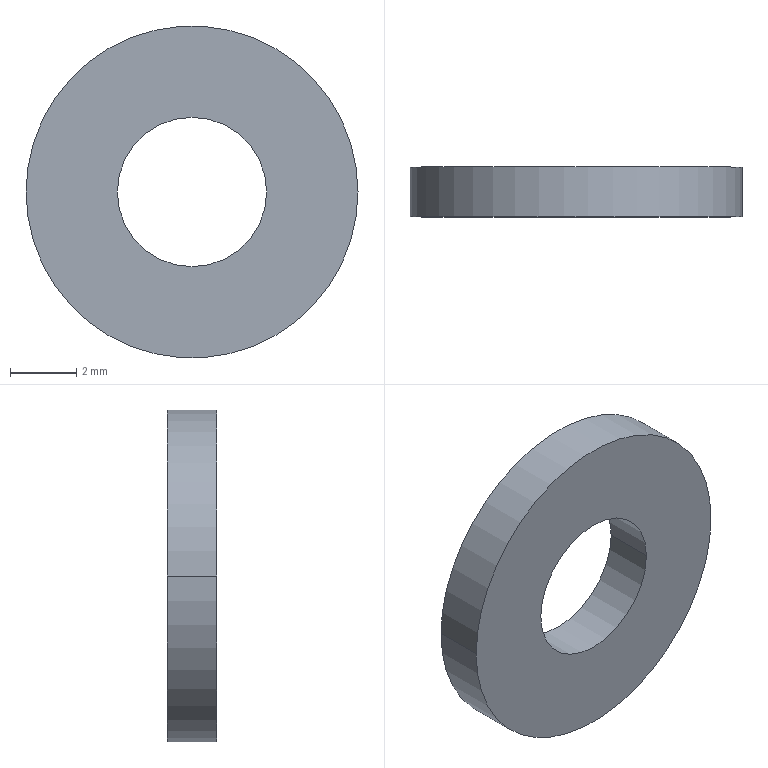Component | SolidWorks | Baffle-2 | 1 solid | 6 faces | box 10 x 1.5 x 10 mm | volume 94 mm3 | cylinder 4 | plane 2 | commonest cylinder face diameters 4.5 x2 10 x2
build123d program:
from build123d import *

# Parameters (mm, degrees)
SKETCH1_R      = 5
SKETCH1_R_2    = 2.25
EXTRUDE1_DEPTH = 1.5


with BuildPart() as part:
    # Sketch1 → Extrude1 (new body)
    with BuildSketch(Plane.XY):
        Circle(SKETCH1_R)
        Circle(SKETCH1_R_2, mode=Mode.SUBTRACT)
    extrude(amount=EXTRUDE1_DEPTH)


solid = part.part

# Placed as in the assembly
solid = solid.moved(Location((43, 41, 5), (90, 0, 0)))
STEP:
#1=COLOUR_RGB('',0.7922,0.8196,0.9333);
#2=FILL_AREA_STYLE_COLOUR('',#1);
#3=FILL_AREA_STYLE('',(#2));
#4=SURFACE_STYLE_FILL_AREA(#3);
#5=SURFACE_SIDE_STYLE('',(#4));
#6=SURFACE_STYLE_USAGE(.BOTH.,#5);
#7=PRESENTATION_STYLE_ASSIGNMENT((#6));
#8=CARTESIAN_POINT('',(1.604,1.555,0.1969));
#9=VERTEX_POINT('',#8);
#10=CARTESIAN_POINT('',(1.781,1.555,0.1969));
#11=VERTEX_POINT('',#10);
#12=CARTESIAN_POINT('',(1.693,1.555,0.1969));
#13=DIRECTION('',(0.,-1.,0.));
#14=DIRECTION('',(1.,0.,0.));
#15=AXIS2_PLACEMENT_3D('',#12,#13,#14);
#16=CIRCLE('',#15,0.08858);
#17=EDGE_CURVE('',#9,#11,#16,.T.);
#18=ORIENTED_EDGE('',*,*,#17,.T.);
#19=CARTESIAN_POINT('',(1.781,1.614,0.1969));
#20=VERTEX_POINT('',#19);
#21=CARTESIAN_POINT('',(1.781,1.555,0.1969));
#22=DIRECTION('',(-0.,1.,-0.));
#23=VECTOR('',#22,39.37);
#24=LINE('',#21,#23);
#25=EDGE_CURVE('',#11,#20,#24,.T.);
#26=ORIENTED_EDGE('',*,*,#25,.T.);
#27=CARTESIAN_POINT('',(1.604,1.614,0.1969));
#28=VERTEX_POINT('',#27);
#29=CARTESIAN_POINT('',(1.693,1.614,0.1969));
#30=DIRECTION('',(0.,-1.,0.));
#31=DIRECTION('',(1.,0.,0.));
#32=AXIS2_PLACEMENT_3D('',#29,#30,#31);
#33=CIRCLE('',#32,0.08858);
#34=EDGE_CURVE('',#28,#20,#33,.T.);
#35=ORIENTED_EDGE('',*,*,#34,.F.);
#36=CARTESIAN_POINT('',(1.604,1.555,0.1969));
#37=DIRECTION('',(-0.,1.,-0.));
#38=VECTOR('',#37,39.37);
#39=LINE('',#36,#38);
#40=EDGE_CURVE('',#9,#28,#39,.T.);
#41=ORIENTED_EDGE('',*,*,#40,.F.);
#42=EDGE_LOOP('',(#18,#26,#35,#41));
#43=FACE_OUTER_BOUND('',#42,.T.);
#44=CARTESIAN_POINT('',(1.693,1.555,0.1969));
#45=DIRECTION('',(-0.,1.,-0.));
#46=DIRECTION('',(-1.,0.,0.));
#47=AXIS2_PLACEMENT_3D('',#44,#45,#46);
#48=CYLINDRICAL_SURFACE('',#47,0.08858);
#49=ADVANCED_FACE('',(#43),#48,.F.);
#50=CARTESIAN_POINT('',(1.89,1.555,0.1969));
#51=VERTEX_POINT('',#50);
#52=CARTESIAN_POINT('',(1.496,1.555,0.1969));
#53=VERTEX_POINT('',#52);
#54=CARTESIAN_POINT('',(1.693,1.555,0.1969));
#55=DIRECTION('',(0.,-1.,0.));
#56=DIRECTION('',(1.,0.,0.));
#57=AXIS2_PLACEMENT_3D('',#54,#55,#56);
#58=CIRCLE('',#57,0.1969);
#59=EDGE_CURVE('',#51,#53,#58,.T.);
#60=ORIENTED_EDGE('',*,*,#59,.F.);
#61=CARTESIAN_POINT('',(1.89,1.614,0.1969));
#62=VERTEX_POINT('',#61);
#63=CARTESIAN_POINT('',(1.89,1.555,0.1969));
#64=DIRECTION('',(-0.,1.,-0.));
#65=VECTOR('',#64,39.37);
#66=LINE('',#63,#65);
#67=EDGE_CURVE('',#51,#62,#66,.T.);
#68=ORIENTED_EDGE('',*,*,#67,.T.);
#69=CARTESIAN_POINT('',(1.496,1.614,0.1969));
#70=VERTEX_POINT('',#69);
#71=CARTESIAN_POINT('',(1.693,1.614,0.1969));
#72=DIRECTION('',(0.,-1.,0.));
#73=DIRECTION('',(1.,0.,0.));
#74=AXIS2_PLACEMENT_3D('',#71,#72,#73);
#75=CIRCLE('',#74,0.1969);
#76=EDGE_CURVE('',#62,#70,#75,.T.);
#77=ORIENTED_EDGE('',*,*,#76,.T.);
#78=CARTESIAN_POINT('',(1.496,1.555,0.1969));
#79=DIRECTION('',(-0.,1.,-0.));
#80=VECTOR('',#79,39.37);
#81=LINE('',#78,#80);
#82=EDGE_CURVE('',#53,#70,#81,.T.);
#83=ORIENTED_EDGE('',*,*,#82,.F.);
#84=EDGE_LOOP('',(#60,#68,#77,#83));
#85=FACE_OUTER_BOUND('',#84,.T.);
#86=CARTESIAN_POINT('',(1.693,1.555,0.1969));
#87=DIRECTION('',(-0.,1.,-0.));
#88=DIRECTION('',(-1.,0.,0.));
#89=AXIS2_PLACEMENT_3D('',#86,#87,#88);
#90=CYLINDRICAL_SURFACE('',#89,0.1969);
#91=ADVANCED_FACE('',(#85),#90,.T.);
#92=CARTESIAN_POINT('',(1.693,1.555,0.1969));
#93=DIRECTION('',(0.,-1.,0.));
#94=DIRECTION('',(1.,0.,0.));
#95=AXIS2_PLACEMENT_3D('',#92,#93,#94);
#96=CIRCLE('',#95,0.1969);
#97=EDGE_CURVE('',#53,#51,#96,.T.);
#98=ORIENTED_EDGE('',*,*,#97,.T.);
#99=ORIENTED_EDGE('',*,*,#59,.T.);
#100=EDGE_LOOP('',(#98,#99));
#101=FACE_OUTER_BOUND('',#100,.T.);
#102=ORIENTED_EDGE('',*,*,#17,.F.);
#103=CARTESIAN_POINT('',(1.693,1.555,0.1969));
#104=DIRECTION('',(0.,-1.,0.));
#105=DIRECTION('',(1.,0.,0.));
#106=AXIS2_PLACEMENT_3D('',#103,#104,#105);
#107=CIRCLE('',#106,0.08858);
#108=EDGE_CURVE('',#11,#9,#107,.T.);
#109=ORIENTED_EDGE('',*,*,#108,.F.);
#110=EDGE_LOOP('',(#102,#109));
#111=FACE_BOUND('',#110,.T.);
#112=CARTESIAN_POINT('',(1.693,1.555,0.1969));
#113=DIRECTION('',(0.,-1.,0.));
#114=DIRECTION('',(1.,0.,-0.));
#115=AXIS2_PLACEMENT_3D('',#112,#113,#114);
#116=PLANE('',#115);
#117=ADVANCED_FACE('',(#101,#111),#116,.T.);
#118=CARTESIAN_POINT('',(1.693,1.614,0.1969));
#119=DIRECTION('',(0.,-1.,0.));
#120=DIRECTION('',(1.,0.,0.));
#121=AXIS2_PLACEMENT_3D('',#118,#119,#120);
#122=CIRCLE('',#121,0.1969);
#123=EDGE_CURVE('',#70,#62,#122,.T.);
#124=ORIENTED_EDGE('',*,*,#123,.F.);
#125=ORIENTED_EDGE('',*,*,#76,.F.);
#126=EDGE_LOOP('',(#124,#125));
#127=FACE_OUTER_BOUND('',#126,.T.);
#128=ORIENTED_EDGE('',*,*,#34,.T.);
#129=CARTESIAN_POINT('',(1.693,1.614,0.1969));
#130=DIRECTION('',(0.,-1.,0.));
#131=DIRECTION('',(1.,0.,0.));
#132=AXIS2_PLACEMENT_3D('',#129,#130,#131);
#133=CIRCLE('',#132,0.08858);
#134=EDGE_CURVE('',#20,#28,#133,.T.);
#135=ORIENTED_EDGE('',*,*,#134,.T.);
#136=EDGE_LOOP('',(#128,#135));
#137=FACE_BOUND('',#136,.T.);
#138=CARTESIAN_POINT('',(1.693,1.614,0.1969));
#139=DIRECTION('',(0.,-1.,0.));
#140=DIRECTION('',(1.,0.,-0.));
#141=AXIS2_PLACEMENT_3D('',#138,#139,#140);
#142=PLANE('',#141);
#143=ADVANCED_FACE('',(#127,#137),#142,.F.);
#144=ORIENTED_EDGE('',*,*,#67,.F.);
#145=ORIENTED_EDGE('',*,*,#97,.F.);
#146=ORIENTED_EDGE('',*,*,#82,.T.);
#147=ORIENTED_EDGE('',*,*,#123,.T.);
#148=EDGE_LOOP('',(#144,#145,#146,#147));
#149=FACE_OUTER_BOUND('',#148,.T.);
#150=CARTESIAN_POINT('',(1.693,1.555,0.1969));
#151=DIRECTION('',(-0.,1.,-0.));
#152=DIRECTION('',(-1.,0.,0.));
#153=AXIS2_PLACEMENT_3D('',#150,#151,#152);
#154=CYLINDRICAL_SURFACE('',#153,0.1969);
#155=ADVANCED_FACE('',(#149),#154,.T.);
#156=ORIENTED_EDGE('',*,*,#25,.F.);
#157=ORIENTED_EDGE('',*,*,#108,.T.);
#158=ORIENTED_EDGE('',*,*,#40,.T.);
#159=ORIENTED_EDGE('',*,*,#134,.F.);
#160=EDGE_LOOP('',(#156,#157,#158,#159));
#161=FACE_OUTER_BOUND('',#160,.T.);
#162=CARTESIAN_POINT('',(1.693,1.555,0.1969));
#163=DIRECTION('',(-0.,1.,-0.));
#164=DIRECTION('',(-1.,0.,0.));
#165=AXIS2_PLACEMENT_3D('',#162,#163,#164);
#166=CYLINDRICAL_SURFACE('',#165,0.08858);
#167=ADVANCED_FACE('',(#161),#166,.F.);
#168=CLOSED_SHELL('',(#49,#91,#117,#143,#155,#167));
#169=MANIFOLD_SOLID_BREP('',#168);
#170=STYLED_ITEM('',(#7),#169);
#171=(LENGTH_UNIT()NAMED_UNIT(*)SI_UNIT($,.METRE.));
#172=LENGTH_MEASURE_WITH_UNIT(LENGTH_MEASURE(0.0254),#171);
#173=DIMENSIONAL_EXPONENTS(1.,0.,0.,0.,0.,0.,0.);
#174=(CONVERSION_BASED_UNIT('',#172)LENGTH_UNIT()NAMED_UNIT(#173));
#175=UNCERTAINTY_MEASURE_WITH_UNIT(LENGTH_MEASURE(0.00001),#174,'','');
#176=(NAMED_UNIT(*)PLANE_ANGLE_UNIT()SI_UNIT($,.RADIAN.));
#177=(NAMED_UNIT(*)SI_UNIT($,.STERADIAN.)SOLID_ANGLE_UNIT());
#178=(GEOMETRIC_REPRESENTATION_CONTEXT(3)GLOBAL_UNCERTAINTY_ASSIGNED_CONTEXT((#175))GLOBAL_UNIT_ASSIGNED_CONTEXT((#174,#176,#177))REPRESENTATION_CONTEXT('',''));
#179=MECHANICAL_DESIGN_GEOMETRIC_PRESENTATION_REPRESENTATION('',(#170),#178);
#180=PRESENTATION_LAYER_ASSIGNMENT('','',(#170));
#181=CARTESIAN_POINT('',(0.,0.,0.));
#182=DIRECTION('',(0.,0.,1.));
#183=DIRECTION('',(1.,0.,0.));
#184=AXIS2_PLACEMENT_3D('',#181,#182,#183);
#185=(LENGTH_UNIT()NAMED_UNIT(*)SI_UNIT($,.METRE.));
#186=LENGTH_MEASURE_WITH_UNIT(LENGTH_MEASURE(0.0254),#185);
#187=DIMENSIONAL_EXPONENTS(1.,0.,0.,0.,0.,0.,0.);
#188=(CONVERSION_BASED_UNIT('',#186)LENGTH_UNIT()NAMED_UNIT(#187));
#189=UNCERTAINTY_MEASURE_WITH_UNIT(LENGTH_MEASURE(0.00001),#188,'','');
#190=(NAMED_UNIT(*)PLANE_ANGLE_UNIT()SI_UNIT($,.RADIAN.));
#191=(NAMED_UNIT(*)SI_UNIT($,.STERADIAN.)SOLID_ANGLE_UNIT());
#192=(GEOMETRIC_REPRESENTATION_CONTEXT(3)GLOBAL_UNCERTAINTY_ASSIGNED_CONTEXT((#189))GLOBAL_UNIT_ASSIGNED_CONTEXT((#188,#190,#191))REPRESENTATION_CONTEXT('',''));
#193=ADVANCED_BREP_SHAPE_REPRESENTATION('',(#169,#184),#192);